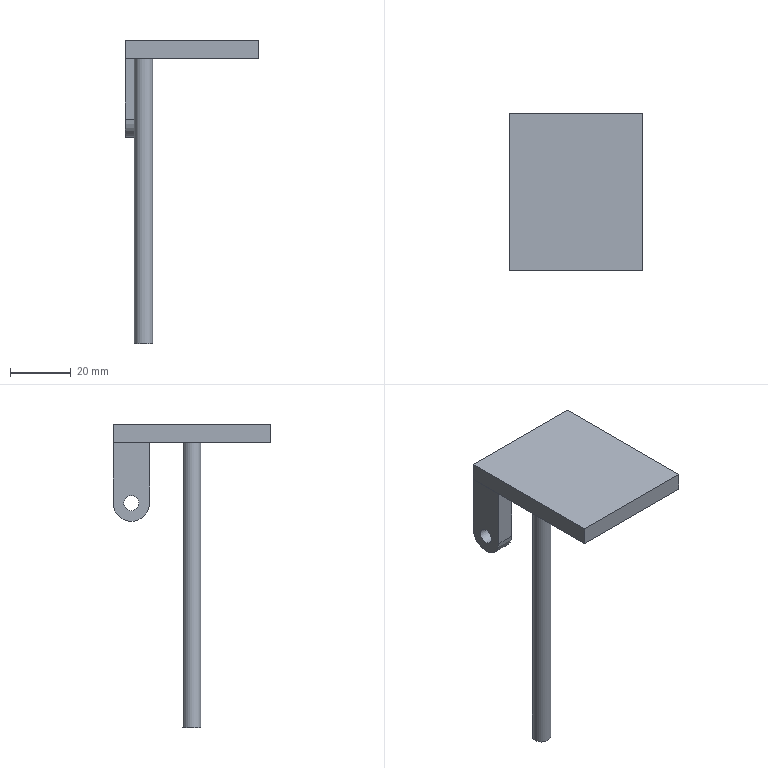Component | NX | PRINT_BLOCK | 3 solids | 16 faces | box 44 x 52.02 x 100 mm | volume 18008 mm3 | plane 13 | cylinder 3 | commonest cylinder face diameters 6 x1 12 x1 5 x1
STEP:
#1=CARTESIAN_POINT('',(0.,0.,0.));
#2=DIRECTION('',(0.,0.,1.));
#3=DIRECTION('',(1.,0.,0.));
#4=AXIS2_PLACEMENT_3D('',#1,#2,#3);
#5=CARTESIAN_POINT('',(44.,110.002,-95.515));
#6=VERTEX_POINT('',#5);
#7=CARTESIAN_POINT('',(47.,110.002,-95.515));
#8=DIRECTION('',(0.,-0.0003321,1.));
#9=DIRECTION('',(-1.,0.,0.));
#10=AXIS2_PLACEMENT_3D('',#7,#8,#9);
#11=CIRCLE('',#10,3.);
#12=CARTESIAN_POINT('',(47.,110.002,-95.515));
#13=DIRECTION('',(0.,-0.0003321,1.));
#14=DIRECTION('',(0.,-1.,-0.0003321));
#15=AXIS2_PLACEMENT_3D('',#12,#13,#14);
#16=CYLINDRICAL_SURFACE('',#15,3.);
#17=CARTESIAN_POINT('',(4.712,0.));
#18=DIRECTION('',(1.,0.));
#19=VECTOR('',#18,1.);
#20=LINE('',#17,#19);
#21=(GEOMETRIC_REPRESENTATION_CONTEXT(2)PARAMETRIC_REPRESENTATION_CONTEXT()REPRESENTATION_CONTEXT('',''));
#22=DEFINITIONAL_REPRESENTATION('',(#20),#21);
#23=PCURVE('',#16,#22);
#24=CARTESIAN_POINT('',(47.,110.002,-95.515));
#25=DIRECTION('',(0.,-0.0003321,1.));
#26=DIRECTION('',(0.,-1.,-0.0003321));
#27=AXIS2_PLACEMENT_3D('',#24,#25,#26);
#28=PLANE('',#27);
#29=CARTESIAN_POINT('',(0.,0.));
#30=DIRECTION('',(0.,-1.));
#31=AXIS2_PLACEMENT_2D('',#29,#30);
#32=CIRCLE('',#31,3.);
#33=(GEOMETRIC_REPRESENTATION_CONTEXT(2)PARAMETRIC_REPRESENTATION_CONTEXT()REPRESENTATION_CONTEXT('',''));
#34=DEFINITIONAL_REPRESENTATION('',(#32),#33);
#35=PCURVE('',#28,#34);
#36=SURFACE_CURVE('',#11,(#23,#35),.PCURVE_S1.);
#37=EDGE_CURVE('',#6,#6,#36,.T.);
#38=ORIENTED_EDGE('',*,*,#37,.T.);
#39=CARTESIAN_POINT('',(44.,109.971,-1.506));
#40=VERTEX_POINT('',#39);
#41=CARTESIAN_POINT('',(44.,110.002,-95.515));
#42=CARTESIAN_POINT('',(44.,109.971,-1.506));
#43=B_SPLINE_CURVE_WITH_KNOTS('',1,(#41,#42),.UNSPECIFIED.,.F.,.F.,(2,2),(0.,94.009),.PIECEWISE_BEZIER_KNOTS.);
#44=CARTESIAN_POINT('',(10.996,0.));
#45=DIRECTION('',(0.,1.));
#46=VECTOR('',#45,1.);
#47=LINE('',#44,#46);
#48=(GEOMETRIC_REPRESENTATION_CONTEXT(2)PARAMETRIC_REPRESENTATION_CONTEXT()REPRESENTATION_CONTEXT('',''));
#49=DEFINITIONAL_REPRESENTATION('',(#47),#48);
#50=PCURVE('',#16,#49);
#51=CARTESIAN_POINT('',(4.712,0.));
#52=DIRECTION('',(0.,1.));
#53=VECTOR('',#52,1.);
#54=LINE('',#51,#53);
#55=(GEOMETRIC_REPRESENTATION_CONTEXT(2)PARAMETRIC_REPRESENTATION_CONTEXT()REPRESENTATION_CONTEXT('',''));
#56=DEFINITIONAL_REPRESENTATION('',(#54),#55);
#57=PCURVE('',#16,#56);
#58=SEAM_CURVE('',#43,(#50,#57),.PCURVE_S1.);
#59=EDGE_CURVE('',#6,#40,#58,.T.);
#60=ORIENTED_EDGE('',*,*,#59,.T.);
#61=CARTESIAN_POINT('',(47.,109.971,-1.506));
#62=DIRECTION('',(0.,-0.0003321,1.));
#63=DIRECTION('',(-1.,0.,0.));
#64=AXIS2_PLACEMENT_3D('',#61,#62,#63);
#65=CIRCLE('',#64,3.);
#66=CARTESIAN_POINT('',(4.712,94.009));
#67=DIRECTION('',(1.,0.));
#68=VECTOR('',#67,1.);
#69=LINE('',#66,#68);
#70=(GEOMETRIC_REPRESENTATION_CONTEXT(2)PARAMETRIC_REPRESENTATION_CONTEXT()REPRESENTATION_CONTEXT('',''));
#71=DEFINITIONAL_REPRESENTATION('',(#69),#70);
#72=PCURVE('',#16,#71);
#73=CARTESIAN_POINT('',(47.,109.971,-1.506));
#74=DIRECTION('',(0.,-0.0003321,1.));
#75=DIRECTION('',(0.,-1.,-0.0003321));
#76=AXIS2_PLACEMENT_3D('',#73,#74,#75);
#77=PLANE('',#76);
#78=CARTESIAN_POINT('',(0.,0.));
#79=DIRECTION('',(0.,-1.));
#80=AXIS2_PLACEMENT_2D('',#78,#79);
#81=CIRCLE('',#80,3.);
#82=(GEOMETRIC_REPRESENTATION_CONTEXT(2)PARAMETRIC_REPRESENTATION_CONTEXT()REPRESENTATION_CONTEXT('',''));
#83=DEFINITIONAL_REPRESENTATION('',(#81),#82);
#84=PCURVE('',#77,#83);
#85=SURFACE_CURVE('',#65,(#72,#84),.PCURVE_S1.);
#86=EDGE_CURVE('',#40,#40,#85,.T.);
#87=ORIENTED_EDGE('',*,*,#86,.F.);
#88=ORIENTED_EDGE('',*,*,#59,.F.);
#89=EDGE_LOOP('',(#38,#60,#87,#88));
#90=FACE_BOUND('',#89,.T.);
#91=ADVANCED_FACE('',(#90),#16,.T.);
#92=ORIENTED_EDGE('',*,*,#37,.F.);
#93=EDGE_LOOP('',(#92));
#94=FACE_BOUND('',#93,.T.);
#95=ADVANCED_FACE('',(#94),#28,.F.);
#96=ORIENTED_EDGE('',*,*,#86,.T.);
#97=EDGE_LOOP('',(#96));
#98=FACE_BOUND('',#97,.T.);
#99=ADVANCED_FACE('',(#98),#77,.T.);
#100=CLOSED_SHELL('',(#91,#95,#99));
#101=MANIFOLD_SOLID_BREP('',#100);
#102=(LENGTH_UNIT()NAMED_UNIT(*)SI_UNIT(.MILLI.,.METRE.));
#103=UNCERTAINTY_MEASURE_WITH_UNIT(LENGTH_MEASURE(0.00001),#102,'','');
#104=(NAMED_UNIT(*)PLANE_ANGLE_UNIT()SI_UNIT($,.RADIAN.));
#105=(NAMED_UNIT(*)SI_UNIT($,.STERADIAN.)SOLID_ANGLE_UNIT());
#106=(GEOMETRIC_REPRESENTATION_CONTEXT(3)GLOBAL_UNCERTAINTY_ASSIGNED_CONTEXT((#103))GLOBAL_UNIT_ASSIGNED_CONTEXT((#102,#104,#105))REPRESENTATION_CONTEXT('',''));
#107=ADVANCED_BREP_SHAPE_REPRESENTATION('',(#4,#101),#106);
#108=CARTESIAN_POINT('',(0.,0.,0.));
#109=DIRECTION('',(0.,0.,1.));
#110=DIRECTION('',(1.,0.,0.));
#111=AXIS2_PLACEMENT_3D('',#108,#109,#110);
#112=CARTESIAN_POINT('',(0.,0.,0.));
#113=DIRECTION('',(0.,0.,1.));
#114=DIRECTION('',(1.,0.,0.));
#115=AXIS2_PLACEMENT_3D('',#112,#113,#114);
#116=CARTESIAN_POINT('',(0.,0.,0.));
#117=DIRECTION('',(0.,0.,1.));
#118=DIRECTION('',(1.,0.,0.));
#119=AXIS2_PLACEMENT_3D('',#116,#117,#118);
#120=(LENGTH_UNIT()NAMED_UNIT(*)SI_UNIT(.MILLI.,.METRE.));
#121=UNCERTAINTY_MEASURE_WITH_UNIT(LENGTH_MEASURE(0.000002),#120,'','');
#122=(NAMED_UNIT(*)PLANE_ANGLE_UNIT()SI_UNIT($,.RADIAN.));
#123=(NAMED_UNIT(*)SI_UNIT($,.STERADIAN.)SOLID_ANGLE_UNIT());
#124=(GEOMETRIC_REPRESENTATION_CONTEXT(3)GLOBAL_UNCERTAINTY_ASSIGNED_CONTEXT((#121))GLOBAL_UNIT_ASSIGNED_CONTEXT((#120,#122,#123))REPRESENTATION_CONTEXT('',''));
#125=SHAPE_REPRESENTATION('',(#4,#111,#115,#119),#124);
#126=ITEM_DEFINED_TRANSFORMATION('','',#4,#111);
#127=(REPRESENTATION_RELATIONSHIP('','',#107,#125)REPRESENTATION_RELATIONSHIP_WITH_TRANSFORMATION(#126)SHAPE_REPRESENTATION_RELATIONSHIP());
#128=CARTESIAN_POINT('',(41.,135.939,-1.497));
#129=VERTEX_POINT('',#128);
#130=CARTESIAN_POINT('',(41.,83.937,-1.515));
#131=VERTEX_POINT('',#130);
#132=CARTESIAN_POINT('',(41.,135.939,-1.497));
#133=DIRECTION('',(0.,-1.,-0.0003321));
#134=VECTOR('',#133,1.);
#135=LINE('',#132,#134);
#136=CARTESIAN_POINT('',(85.,135.939,-1.497));
#137=DIRECTION('',(0.,0.0003321,-1.));
#138=DIRECTION('',(0.,1.,0.0003321));
#139=AXIS2_PLACEMENT_3D('',#136,#137,#138);
#140=PLANE('',#139);
#141=CARTESIAN_POINT('',(0.,-44.));
#142=DIRECTION('',(-1.,0.));
#143=VECTOR('',#142,1.);
#144=LINE('',#141,#143);
#145=(GEOMETRIC_REPRESENTATION_CONTEXT(2)PARAMETRIC_REPRESENTATION_CONTEXT()REPRESENTATION_CONTEXT('',''));
#146=DEFINITIONAL_REPRESENTATION('',(#144),#145);
#147=PCURVE('',#140,#146);
#148=CARTESIAN_POINT('',(41.,199.9,58.545));
#149=DIRECTION('',(-1.,0.,0.));
#150=DIRECTION('',(0.,1.,0.0006642));
#151=AXIS2_PLACEMENT_3D('',#148,#149,#150);
#152=PLANE('',#151);
#153=CARTESIAN_POINT('',(-64.,60.));
#154=DIRECTION('',(-1.,-0.0003321));
#155=VECTOR('',#154,1.);
#156=LINE('',#153,#155);
#157=(GEOMETRIC_REPRESENTATION_CONTEXT(2)PARAMETRIC_REPRESENTATION_CONTEXT()REPRESENTATION_CONTEXT('',''));
#158=DEFINITIONAL_REPRESENTATION('',(#156),#157);
#159=PCURVE('',#152,#158);
#160=SURFACE_CURVE('',#135,(#147,#159),.PCURVE_S1.);
#161=EDGE_CURVE('',#129,#131,#160,.T.);
#162=ORIENTED_EDGE('',*,*,#161,.F.);
#163=CARTESIAN_POINT('',(85.,135.939,-1.497));
#164=VERTEX_POINT('',#163);
#165=CARTESIAN_POINT('',(85.,135.939,-1.497));
#166=DIRECTION('',(-1.,0.,0.));
#167=VECTOR('',#166,1.);
#168=LINE('',#165,#167);
#169=CARTESIAN_POINT('',(0.,0.));
#170=DIRECTION('',(0.,-1.));
#171=VECTOR('',#170,1.);
#172=LINE('',#169,#171);
#173=(GEOMETRIC_REPRESENTATION_CONTEXT(2)PARAMETRIC_REPRESENTATION_CONTEXT()REPRESENTATION_CONTEXT('',''));
#174=DEFINITIONAL_REPRESENTATION('',(#172),#173);
#175=PCURVE('',#140,#174);
#176=CARTESIAN_POINT('',(85.,135.937,4.485));
#177=DIRECTION('',(0.,1.,0.0003321));
#178=DIRECTION('',(0.,-0.0003321,1.));
#179=AXIS2_PLACEMENT_3D('',#176,#177,#178);
#180=PLANE('',#179);
#181=CARTESIAN_POINT('',(-5.983,0.));
#182=DIRECTION('',(0.,-1.));
#183=VECTOR('',#182,1.);
#184=LINE('',#181,#183);
#185=(GEOMETRIC_REPRESENTATION_CONTEXT(2)PARAMETRIC_REPRESENTATION_CONTEXT()REPRESENTATION_CONTEXT('',''));
#186=DEFINITIONAL_REPRESENTATION('',(#184),#185);
#187=PCURVE('',#180,#186);
#188=SURFACE_CURVE('',#168,(#175,#187),.PCURVE_S1.);
#189=EDGE_CURVE('',#164,#129,#188,.T.);
#190=ORIENTED_EDGE('',*,*,#189,.F.);
#191=CARTESIAN_POINT('',(85.,83.937,-1.515));
#192=VERTEX_POINT('',#191);
#193=CARTESIAN_POINT('',(85.,135.939,-1.497));
#194=DIRECTION('',(0.,-1.,-0.0003321));
#195=VECTOR('',#194,1.);
#196=LINE('',#193,#195);
#197=CARTESIAN_POINT('',(0.,0.));
#198=DIRECTION('',(-1.,0.));
#199=VECTOR('',#198,1.);
#200=LINE('',#197,#199);
#201=(GEOMETRIC_REPRESENTATION_CONTEXT(2)PARAMETRIC_REPRESENTATION_CONTEXT()REPRESENTATION_CONTEXT('',''));
#202=DEFINITIONAL_REPRESENTATION('',(#200),#201);
#203=PCURVE('',#140,#202);
#204=CARTESIAN_POINT('',(85.,199.9,58.545));
#205=DIRECTION('',(-1.,0.,0.));
#206=DIRECTION('',(0.,1.,0.0006642));
#207=AXIS2_PLACEMENT_3D('',#204,#205,#206);
#208=PLANE('',#207);
#209=CARTESIAN_POINT('',(-64.,60.));
#210=DIRECTION('',(-1.,-0.0003321));
#211=VECTOR('',#210,1.);
#212=LINE('',#209,#211);
#213=(GEOMETRIC_REPRESENTATION_CONTEXT(2)PARAMETRIC_REPRESENTATION_CONTEXT()REPRESENTATION_CONTEXT('',''));
#214=DEFINITIONAL_REPRESENTATION('',(#212),#213);
#215=PCURVE('',#208,#214);
#216=SURFACE_CURVE('',#196,(#203,#215),.PCURVE_S1.);
#217=EDGE_CURVE('',#164,#192,#216,.T.);
#218=ORIENTED_EDGE('',*,*,#217,.T.);
#219=CARTESIAN_POINT('',(85.,83.937,-1.515));
#220=DIRECTION('',(-1.,0.,0.));
#221=VECTOR('',#220,1.);
#222=LINE('',#219,#221);
#223=CARTESIAN_POINT('',(-52.002,0.));
#224=DIRECTION('',(0.,-1.));
#225=VECTOR('',#224,1.);
#226=LINE('',#223,#225);
#227=(GEOMETRIC_REPRESENTATION_CONTEXT(2)PARAMETRIC_REPRESENTATION_CONTEXT()REPRESENTATION_CONTEXT('',''));
#228=DEFINITIONAL_REPRESENTATION('',(#226),#227);
#229=PCURVE('',#140,#228);
#230=CARTESIAN_POINT('',(85.,83.937,-1.515));
#231=DIRECTION('',(0.,-1.,-0.0003321));
#232=DIRECTION('',(0.,0.0003321,-1.));
#233=AXIS2_PLACEMENT_3D('',#230,#231,#232);
#234=PLANE('',#233);
#235=CARTESIAN_POINT('',(0.,0.));
#236=DIRECTION('',(0.,-1.));
#237=VECTOR('',#236,1.);
#238=LINE('',#235,#237);
#239=(GEOMETRIC_REPRESENTATION_CONTEXT(2)PARAMETRIC_REPRESENTATION_CONTEXT()REPRESENTATION_CONTEXT('',''));
#240=DEFINITIONAL_REPRESENTATION('',(#238),#239);
#241=PCURVE('',#234,#240);
#242=SURFACE_CURVE('',#222,(#229,#241),.PCURVE_S1.);
#243=EDGE_CURVE('',#192,#131,#242,.T.);
#244=ORIENTED_EDGE('',*,*,#243,.T.);
#245=EDGE_LOOP('',(#162,#190,#218,#244));
#246=FACE_BOUND('',#245,.T.);
#247=ADVANCED_FACE('',(#246),#140,.T.);
#248=CARTESIAN_POINT('',(41.,83.935,4.468));
#249=VERTEX_POINT('',#248);
#250=CARTESIAN_POINT('',(41.,83.937,-1.515));
#251=DIRECTION('',(0.,-0.0003321,1.));
#252=VECTOR('',#251,1.);
#253=LINE('',#250,#252);
#254=CARTESIAN_POINT('',(0.,-44.));
#255=DIRECTION('',(-1.,0.));
#256=VECTOR('',#255,1.);
#257=LINE('',#254,#256);
#258=(GEOMETRIC_REPRESENTATION_CONTEXT(2)PARAMETRIC_REPRESENTATION_CONTEXT()REPRESENTATION_CONTEXT('',''));
#259=DEFINITIONAL_REPRESENTATION('',(#257),#258);
#260=PCURVE('',#234,#259);
#261=CARTESIAN_POINT('',(-116.002,59.983));
#262=DIRECTION('',(0.0003321,-1.));
#263=VECTOR('',#262,1.);
#264=LINE('',#261,#263);
#265=(GEOMETRIC_REPRESENTATION_CONTEXT(2)PARAMETRIC_REPRESENTATION_CONTEXT()REPRESENTATION_CONTEXT('',''));
#266=DEFINITIONAL_REPRESENTATION('',(#264),#265);
#267=PCURVE('',#152,#266);
#268=SURFACE_CURVE('',#253,(#260,#267),.PCURVE_S1.);
#269=EDGE_CURVE('',#131,#249,#268,.T.);
#270=ORIENTED_EDGE('',*,*,#269,.F.);
#271=ORIENTED_EDGE('',*,*,#243,.F.);
#272=CARTESIAN_POINT('',(85.,83.935,4.468));
#273=VERTEX_POINT('',#272);
#274=CARTESIAN_POINT('',(85.,83.937,-1.515));
#275=DIRECTION('',(0.,-0.0003321,1.));
#276=VECTOR('',#275,1.);
#277=LINE('',#274,#276);
#278=CARTESIAN_POINT('',(0.,0.));
#279=DIRECTION('',(-1.,0.));
#280=VECTOR('',#279,1.);
#281=LINE('',#278,#280);
#282=(GEOMETRIC_REPRESENTATION_CONTEXT(2)PARAMETRIC_REPRESENTATION_CONTEXT()REPRESENTATION_CONTEXT('',''));
#283=DEFINITIONAL_REPRESENTATION('',(#281),#282);
#284=PCURVE('',#234,#283);
#285=CARTESIAN_POINT('',(-116.002,59.983));
#286=DIRECTION('',(0.0003321,-1.));
#287=VECTOR('',#286,1.);
#288=LINE('',#285,#287);
#289=(GEOMETRIC_REPRESENTATION_CONTEXT(2)PARAMETRIC_REPRESENTATION_CONTEXT()REPRESENTATION_CONTEXT('',''));
#290=DEFINITIONAL_REPRESENTATION('',(#288),#289);
#291=PCURVE('',#208,#290);
#292=SURFACE_CURVE('',#277,(#284,#291),.PCURVE_S1.);
#293=EDGE_CURVE('',#192,#273,#292,.T.);
#294=ORIENTED_EDGE('',*,*,#293,.T.);
#295=CARTESIAN_POINT('',(85.,83.935,4.468));
#296=DIRECTION('',(-1.,0.,0.));
#297=VECTOR('',#296,1.);
#298=LINE('',#295,#297);
#299=CARTESIAN_POINT('',(-5.983,0.));
#300=DIRECTION('',(0.,-1.));
#301=VECTOR('',#300,1.);
#302=LINE('',#299,#301);
#303=(GEOMETRIC_REPRESENTATION_CONTEXT(2)PARAMETRIC_REPRESENTATION_CONTEXT()REPRESENTATION_CONTEXT('',''));
#304=DEFINITIONAL_REPRESENTATION('',(#302),#303);
#305=PCURVE('',#234,#304);
#306=CARTESIAN_POINT('',(85.,83.935,4.468));
#307=DIRECTION('',(0.,-0.0003321,1.));
#308=DIRECTION('',(0.,-1.,-0.0003321));
#309=AXIS2_PLACEMENT_3D('',#306,#307,#308);
#310=PLANE('',#309);
#311=CARTESIAN_POINT('',(0.,0.));
#312=DIRECTION('',(0.,-1.));
#313=VECTOR('',#312,1.);
#314=LINE('',#311,#313);
#315=(GEOMETRIC_REPRESENTATION_CONTEXT(2)PARAMETRIC_REPRESENTATION_CONTEXT()REPRESENTATION_CONTEXT('',''));
#316=DEFINITIONAL_REPRESENTATION('',(#314),#315);
#317=PCURVE('',#310,#316);
#318=SURFACE_CURVE('',#298,(#305,#317),.PCURVE_S1.);
#319=EDGE_CURVE('',#273,#249,#318,.T.);
#320=ORIENTED_EDGE('',*,*,#319,.T.);
#321=EDGE_LOOP('',(#270,#271,#294,#320));
#322=FACE_BOUND('',#321,.T.);
#323=ADVANCED_FACE('',(#322),#234,.T.);
#324=CARTESIAN_POINT('',(41.,135.937,4.485));
#325=VERTEX_POINT('',#324);
#326=CARTESIAN_POINT('',(41.,83.935,4.468));
#327=DIRECTION('',(0.,1.,0.0003321));
#328=VECTOR('',#327,1.);
#329=LINE('',#326,#328);
#330=CARTESIAN_POINT('',(0.,-44.));
#331=DIRECTION('',(-1.,0.));
#332=VECTOR('',#331,1.);
#333=LINE('',#330,#332);
#334=(GEOMETRIC_REPRESENTATION_CONTEXT(2)PARAMETRIC_REPRESENTATION_CONTEXT()REPRESENTATION_CONTEXT('',''));
#335=DEFINITIONAL_REPRESENTATION('',(#333),#334);
#336=PCURVE('',#310,#335);
#337=CARTESIAN_POINT('',(-116.,54.));
#338=DIRECTION('',(1.,0.0003321));
#339=VECTOR('',#338,1.);
#340=LINE('',#337,#339);
#341=(GEOMETRIC_REPRESENTATION_CONTEXT(2)PARAMETRIC_REPRESENTATION_CONTEXT()REPRESENTATION_CONTEXT('',''));
#342=DEFINITIONAL_REPRESENTATION('',(#340),#341);
#343=PCURVE('',#152,#342);
#344=SURFACE_CURVE('',#329,(#336,#343),.PCURVE_S1.);
#345=EDGE_CURVE('',#249,#325,#344,.T.);
#346=ORIENTED_EDGE('',*,*,#345,.F.);
#347=ORIENTED_EDGE('',*,*,#319,.F.);
#348=CARTESIAN_POINT('',(85.,135.937,4.485));
#349=VERTEX_POINT('',#348);
#350=CARTESIAN_POINT('',(85.,83.935,4.468));
#351=DIRECTION('',(0.,1.,0.0003321));
#352=VECTOR('',#351,1.);
#353=LINE('',#350,#352);
#354=CARTESIAN_POINT('',(0.,0.));
#355=DIRECTION('',(-1.,0.));
#356=VECTOR('',#355,1.);
#357=LINE('',#354,#356);
#358=(GEOMETRIC_REPRESENTATION_CONTEXT(2)PARAMETRIC_REPRESENTATION_CONTEXT()REPRESENTATION_CONTEXT('',''));
#359=DEFINITIONAL_REPRESENTATION('',(#357),#358);
#360=PCURVE('',#310,#359);
#361=CARTESIAN_POINT('',(-116.,54.));
#362=DIRECTION('',(1.,0.0003321));
#363=VECTOR('',#362,1.);
#364=LINE('',#361,#363);
#365=(GEOMETRIC_REPRESENTATION_CONTEXT(2)PARAMETRIC_REPRESENTATION_CONTEXT()REPRESENTATION_CONTEXT('',''));
#366=DEFINITIONAL_REPRESENTATION('',(#364),#365);
#367=PCURVE('',#208,#366);
#368=SURFACE_CURVE('',#353,(#360,#367),.PCURVE_S1.);
#369=EDGE_CURVE('',#273,#349,#368,.T.);
#370=ORIENTED_EDGE('',*,*,#369,.T.);
#371=CARTESIAN_POINT('',(85.,135.937,4.485));
#372=DIRECTION('',(-1.,0.,0.));
#373=VECTOR('',#372,1.);
#374=LINE('',#371,#373);
#375=CARTESIAN_POINT('',(-52.002,0.));
#376=DIRECTION('',(0.,-1.));
#377=VECTOR('',#376,1.);
#378=LINE('',#375,#377);
#379=(GEOMETRIC_REPRESENTATION_CONTEXT(2)PARAMETRIC_REPRESENTATION_CONTEXT()REPRESENTATION_CONTEXT('',''));
#380=DEFINITIONAL_REPRESENTATION('',(#378),#379);
#381=PCURVE('',#310,#380);
#382=CARTESIAN_POINT('',(0.,0.));
#383=DIRECTION('',(0.,-1.));
#384=VECTOR('',#383,1.);
#385=LINE('',#382,#384);
#386=(GEOMETRIC_REPRESENTATION_CONTEXT(2)PARAMETRIC_REPRESENTATION_CONTEXT()REPRESENTATION_CONTEXT('',''));
#387=DEFINITIONAL_REPRESENTATION('',(#385),#386);
#388=PCURVE('',#180,#387);
#389=SURFACE_CURVE('',#374,(#381,#388),.PCURVE_S1.);
#390=EDGE_CURVE('',#349,#325,#389,.T.);
#391=ORIENTED_EDGE('',*,*,#390,.T.);
#392=EDGE_LOOP('',(#346,#347,#370,#391));
#393=FACE_BOUND('',#392,.T.);
#394=ADVANCED_FACE('',(#393),#310,.T.);
#395=CARTESIAN_POINT('',(41.,135.937,4.485));
#396=DIRECTION('',(0.,0.0003321,-1.));
#397=VECTOR('',#396,1.);
#398=LINE('',#395,#397);
#399=CARTESIAN_POINT('',(0.,-44.));
#400=DIRECTION('',(-1.,0.));
#401=VECTOR('',#400,1.);
#402=LINE('',#399,#401);
#403=(GEOMETRIC_REPRESENTATION_CONTEXT(2)PARAMETRIC_REPRESENTATION_CONTEXT()REPRESENTATION_CONTEXT('',''));
#404=DEFINITIONAL_REPRESENTATION('',(#402),#403);
#405=PCURVE('',#180,#404);
#406=CARTESIAN_POINT('',(-63.998,54.017));
#407=DIRECTION('',(-0.0003321,1.));
#408=VECTOR('',#407,1.);
#409=LINE('',#406,#408);
#410=(GEOMETRIC_REPRESENTATION_CONTEXT(2)PARAMETRIC_REPRESENTATION_CONTEXT()REPRESENTATION_CONTEXT('',''));
#411=DEFINITIONAL_REPRESENTATION('',(#409),#410);
#412=PCURVE('',#152,#411);
#413=SURFACE_CURVE('',#398,(#405,#412),.PCURVE_S1.);
#414=EDGE_CURVE('',#325,#129,#413,.T.);
#415=ORIENTED_EDGE('',*,*,#414,.F.);
#416=ORIENTED_EDGE('',*,*,#390,.F.);
#417=CARTESIAN_POINT('',(85.,135.937,4.485));
#418=DIRECTION('',(0.,0.0003321,-1.));
#419=VECTOR('',#418,1.);
#420=LINE('',#417,#419);
#421=CARTESIAN_POINT('',(0.,0.));
#422=DIRECTION('',(-1.,0.));
#423=VECTOR('',#422,1.);
#424=LINE('',#421,#423);
#425=(GEOMETRIC_REPRESENTATION_CONTEXT(2)PARAMETRIC_REPRESENTATION_CONTEXT()REPRESENTATION_CONTEXT('',''));
#426=DEFINITIONAL_REPRESENTATION('',(#424),#425);
#427=PCURVE('',#180,#426);
#428=CARTESIAN_POINT('',(-63.998,54.017));
#429=DIRECTION('',(-0.0003321,1.));
#430=VECTOR('',#429,1.);
#431=LINE('',#428,#430);
#432=(GEOMETRIC_REPRESENTATION_CONTEXT(2)PARAMETRIC_REPRESENTATION_CONTEXT()REPRESENTATION_CONTEXT('',''));
#433=DEFINITIONAL_REPRESENTATION('',(#431),#432);
#434=PCURVE('',#208,#433);
#435=SURFACE_CURVE('',#420,(#427,#434),.PCURVE_S1.);
#436=EDGE_CURVE('',#349,#164,#435,.T.);
#437=ORIENTED_EDGE('',*,*,#436,.T.);
#438=ORIENTED_EDGE('',*,*,#189,.T.);
#439=EDGE_LOOP('',(#415,#416,#437,#438));
#440=FACE_BOUND('',#439,.T.);
#441=ADVANCED_FACE('',(#440),#180,.T.);
#442=ORIENTED_EDGE('',*,*,#217,.F.);
#443=ORIENTED_EDGE('',*,*,#436,.F.);
#444=ORIENTED_EDGE('',*,*,#369,.F.);
#445=ORIENTED_EDGE('',*,*,#293,.F.);
#446=EDGE_LOOP('',(#442,#443,#444,#445));
#447=FACE_BOUND('',#446,.T.);
#448=ADVANCED_FACE('',(#447),#208,.F.);
#449=ORIENTED_EDGE('',*,*,#161,.T.);
#450=ORIENTED_EDGE('',*,*,#269,.T.);
#451=ORIENTED_EDGE('',*,*,#345,.T.);
#452=ORIENTED_EDGE('',*,*,#414,.T.);
#453=EDGE_LOOP('',(#449,#450,#451,#452));
#454=FACE_BOUND('',#453,.T.);
#455=ADVANCED_FACE('',(#454),#152,.T.);
#456=CLOSED_SHELL('',(#247,#323,#394,#441,#448,#455));
#457=MANIFOLD_SOLID_BREP('',#456);
#458=(LENGTH_UNIT()NAMED_UNIT(*)SI_UNIT(.MILLI.,.METRE.));
#459=UNCERTAINTY_MEASURE_WITH_UNIT(LENGTH_MEASURE(0.0000001),#458,'','');
#460=(NAMED_UNIT(*)PLANE_ANGLE_UNIT()SI_UNIT($,.RADIAN.));
#461=(NAMED_UNIT(*)SI_UNIT($,.STERADIAN.)SOLID_ANGLE_UNIT());
#462=(GEOMETRIC_REPRESENTATION_CONTEXT(3)GLOBAL_UNCERTAINTY_ASSIGNED_CONTEXT((#459))GLOBAL_UNIT_ASSIGNED_CONTEXT((#458,#460,#461))REPRESENTATION_CONTEXT('',''));
#463=ADVANCED_BREP_SHAPE_REPRESENTATION('',(#4,#457),#462);
#464=ITEM_DEFINED_TRANSFORMATION('','',#4,#115);
#465=(REPRESENTATION_RELATIONSHIP('','',#463,#125)REPRESENTATION_RELATIONSHIP_WITH_TRANSFORMATION(#464)SHAPE_REPRESENTATION_RELATIONSHIP());
#466=CARTESIAN_POINT('',(47.,135.946,-21.217));
#467=VERTEX_POINT('',#466);
#468=CARTESIAN_POINT('',(47.,123.953,-21.501));
#469=VERTEX_POINT('',#468);
#470=CARTESIAN_POINT('',(47.,129.953,-21.501));
#471=DIRECTION('',(-1.,0.,0.));
#472=DIRECTION('',(0.,0.0003321,-1.));
#473=AXIS2_PLACEMENT_3D('',#470,#471,#472);
#474=CIRCLE('',#473,6.);
#475=CARTESIAN_POINT('',(41.,129.953,-21.501));
#476=DIRECTION('',(1.,0.,0.));
#477=DIRECTION('',(0.,-1.,-0.0006642));
#478=AXIS2_PLACEMENT_3D('',#475,#476,#477);
#479=CYLINDRICAL_SURFACE('',#478,6.);
#480=CARTESIAN_POINT('',(7.854,6.));
#481=DIRECTION('',(-1.,0.));
#482=VECTOR('',#481,1.);
#483=LINE('',#480,#482);
#484=(GEOMETRIC_REPRESENTATION_CONTEXT(2)PARAMETRIC_REPRESENTATION_CONTEXT()REPRESENTATION_CONTEXT('',''));
#485=DEFINITIONAL_REPRESENTATION('',(#483),#484);
#486=PCURVE('',#479,#485);
#487=CARTESIAN_POINT('',(47.,129.953,-21.501));
#488=DIRECTION('',(-1.,0.,0.));
#489=DIRECTION('',(0.,1.,0.0006642));
#490=AXIS2_PLACEMENT_3D('',#487,#488,#489);
#491=PLANE('',#490);
#492=CARTESIAN_POINT('',(0.,0.));
#493=DIRECTION('',(-0.0003321,1.));
#494=AXIS2_PLACEMENT_2D('',#492,#493);
#495=CIRCLE('',#494,6.);
#496=(GEOMETRIC_REPRESENTATION_CONTEXT(2)PARAMETRIC_REPRESENTATION_CONTEXT()REPRESENTATION_CONTEXT('',''));
#497=DEFINITIONAL_REPRESENTATION('',(#495),#496);
#498=PCURVE('',#491,#497);
#499=SURFACE_CURVE('',#474,(#486,#498),.PCURVE_S1.);
#500=EDGE_CURVE('',#467,#469,#499,.T.);
#501=ORIENTED_EDGE('',*,*,#500,.T.);
#502=CARTESIAN_POINT('',(41.,123.953,-21.501));
#503=VERTEX_POINT('',#502);
#504=CARTESIAN_POINT('',(41.,123.953,-21.501));
#505=DIRECTION('',(1.,0.,0.));
#506=VECTOR('',#505,1.);
#507=LINE('',#504,#506);
#508=CARTESIAN_POINT('',(-0.0006903,0.));
#509=DIRECTION('',(0.,1.));
#510=VECTOR('',#509,1.);
#511=LINE('',#508,#510);
#512=(GEOMETRIC_REPRESENTATION_CONTEXT(2)PARAMETRIC_REPRESENTATION_CONTEXT()REPRESENTATION_CONTEXT('',''));
#513=DEFINITIONAL_REPRESENTATION('',(#511),#512);
#514=PCURVE('',#479,#513);
#515=CARTESIAN_POINT('',(41.,123.953,-21.501));
#516=DIRECTION('',(0.,1.,0.0003321));
#517=DIRECTION('',(0.,-0.0003321,1.));
#518=AXIS2_PLACEMENT_3D('',#515,#516,#517);
#519=PLANE('',#518);
#520=CARTESIAN_POINT('',(-0.,0.));
#521=DIRECTION('',(0.,1.));
#522=VECTOR('',#521,1.);
#523=LINE('',#520,#522);
#524=(GEOMETRIC_REPRESENTATION_CONTEXT(2)PARAMETRIC_REPRESENTATION_CONTEXT()REPRESENTATION_CONTEXT('',''));
#525=DEFINITIONAL_REPRESENTATION('',(#523),#524);
#526=PCURVE('',#519,#525);
#527=SURFACE_CURVE('',#507,(#514,#526),.PCURVE_S1.);
#528=EDGE_CURVE('',#503,#469,#527,.T.);
#529=ORIENTED_EDGE('',*,*,#528,.F.);
#530=CARTESIAN_POINT('',(41.,135.946,-21.217));
#531=VERTEX_POINT('',#530);
#532=CARTESIAN_POINT('',(41.,129.953,-21.501));
#533=DIRECTION('',(-1.,0.,0.));
#534=DIRECTION('',(0.,0.0003321,-1.));
#535=AXIS2_PLACEMENT_3D('',#532,#533,#534);
#536=CIRCLE('',#535,6.);
#537=CARTESIAN_POINT('',(7.854,0.));
#538=DIRECTION('',(-1.,0.));
#539=VECTOR('',#538,1.);
#540=LINE('',#537,#539);
#541=(GEOMETRIC_REPRESENTATION_CONTEXT(2)PARAMETRIC_REPRESENTATION_CONTEXT()REPRESENTATION_CONTEXT('',''));
#542=DEFINITIONAL_REPRESENTATION('',(#540),#541);
#543=PCURVE('',#479,#542);
#544=CARTESIAN_POINT('',(41.,129.953,-21.501));
#545=DIRECTION('',(-1.,0.,0.));
#546=DIRECTION('',(0.,1.,0.0006642));
#547=AXIS2_PLACEMENT_3D('',#544,#545,#546);
#548=PLANE('',#547);
#549=CARTESIAN_POINT('',(0.,0.));
#550=DIRECTION('',(-0.0003321,1.));
#551=AXIS2_PLACEMENT_2D('',#549,#550);
#552=CIRCLE('',#551,6.);
#553=(GEOMETRIC_REPRESENTATION_CONTEXT(2)PARAMETRIC_REPRESENTATION_CONTEXT()REPRESENTATION_CONTEXT('',''));
#554=DEFINITIONAL_REPRESENTATION('',(#552),#553);
#555=PCURVE('',#548,#554);
#556=SURFACE_CURVE('',#536,(#543,#555),.PCURVE_S1.);
#557=EDGE_CURVE('',#531,#503,#556,.T.);
#558=ORIENTED_EDGE('',*,*,#557,.F.);
#559=CARTESIAN_POINT('',(41.,135.946,-21.217));
#560=DIRECTION('',(1.,0.,0.));
#561=VECTOR('',#560,1.);
#562=LINE('',#559,#561);
#563=CARTESIAN_POINT('',(3.188,0.));
#564=DIRECTION('',(0.,1.));
#565=VECTOR('',#564,1.);
#566=LINE('',#563,#565);
#567=(GEOMETRIC_REPRESENTATION_CONTEXT(2)PARAMETRIC_REPRESENTATION_CONTEXT()REPRESENTATION_CONTEXT('',''));
#568=DEFINITIONAL_REPRESENTATION('',(#566),#567);
#569=PCURVE('',#479,#568);
#570=CARTESIAN_POINT('',(41.,135.939,-1.497));
#571=DIRECTION('',(0.,-1.,-0.0003321));
#572=DIRECTION('',(0.,0.0003321,-1.));
#573=AXIS2_PLACEMENT_3D('',#570,#571,#572);
#574=PLANE('',#573);
#575=CARTESIAN_POINT('',(19.72,0.));
#576=DIRECTION('',(0.,1.));
#577=VECTOR('',#576,1.);
#578=LINE('',#575,#577);
#579=(GEOMETRIC_REPRESENTATION_CONTEXT(2)PARAMETRIC_REPRESENTATION_CONTEXT()REPRESENTATION_CONTEXT('',''));
#580=DEFINITIONAL_REPRESENTATION('',(#578),#579);
#581=PCURVE('',#574,#580);
#582=SURFACE_CURVE('',#562,(#569,#581),.PCURVE_S1.);
#583=EDGE_CURVE('',#531,#467,#582,.T.);
#584=ORIENTED_EDGE('',*,*,#583,.T.);
#585=EDGE_LOOP('',(#501,#529,#558,#584));
#586=FACE_BOUND('',#585,.T.);
#587=ADVANCED_FACE('',(#586),#479,.T.);
#588=CARTESIAN_POINT('',(47.,123.946,-1.501));
#589=VERTEX_POINT('',#588);
#590=CARTESIAN_POINT('',(47.,123.953,-21.501));
#591=DIRECTION('',(0.,-0.0003321,1.));
#592=VECTOR('',#591,1.);
#593=LINE('',#590,#592);
#594=CARTESIAN_POINT('',(0.,6.));
#595=DIRECTION('',(1.,0.));
#596=VECTOR('',#595,1.);
#597=LINE('',#594,#596);
#598=(GEOMETRIC_REPRESENTATION_CONTEXT(2)PARAMETRIC_REPRESENTATION_CONTEXT()REPRESENTATION_CONTEXT('',''));
#599=DEFINITIONAL_REPRESENTATION('',(#597),#598);
#600=PCURVE('',#519,#599);
#601=CARTESIAN_POINT('',(-6.,-0.004142));
#602=DIRECTION('',(0.0003321,-1.));
#603=VECTOR('',#602,1.);
#604=LINE('',#601,#603);
#605=(GEOMETRIC_REPRESENTATION_CONTEXT(2)PARAMETRIC_REPRESENTATION_CONTEXT()REPRESENTATION_CONTEXT('',''));
#606=DEFINITIONAL_REPRESENTATION('',(#604),#605);
#607=PCURVE('',#491,#606);
#608=SURFACE_CURVE('',#593,(#600,#607),.PCURVE_S1.);
#609=EDGE_CURVE('',#469,#589,#608,.T.);
#610=ORIENTED_EDGE('',*,*,#609,.T.);
#611=CARTESIAN_POINT('',(41.,123.946,-1.501));
#612=VERTEX_POINT('',#611);
#613=CARTESIAN_POINT('',(41.,123.946,-1.501));
#614=DIRECTION('',(1.,0.,0.));
#615=VECTOR('',#614,1.);
#616=LINE('',#613,#615);
#617=CARTESIAN_POINT('',(20.,0.));
#618=DIRECTION('',(0.,1.));
#619=VECTOR('',#618,1.);
#620=LINE('',#617,#619);
#621=(GEOMETRIC_REPRESENTATION_CONTEXT(2)PARAMETRIC_REPRESENTATION_CONTEXT()REPRESENTATION_CONTEXT('',''));
#622=DEFINITIONAL_REPRESENTATION('',(#620),#621);
#623=PCURVE('',#519,#622);
#624=CARTESIAN_POINT('',(41.,123.946,-1.501));
#625=DIRECTION('',(0.,0.0003321,-1.));
#626=DIRECTION('',(0.,1.,0.0003321));
#627=AXIS2_PLACEMENT_3D('',#624,#625,#626);
#628=PLANE('',#627);
#629=CARTESIAN_POINT('',(0.,0.));
#630=DIRECTION('',(0.,1.));
#631=VECTOR('',#630,1.);
#632=LINE('',#629,#631);
#633=(GEOMETRIC_REPRESENTATION_CONTEXT(2)PARAMETRIC_REPRESENTATION_CONTEXT()REPRESENTATION_CONTEXT('',''));
#634=DEFINITIONAL_REPRESENTATION('',(#632),#633);
#635=PCURVE('',#628,#634);
#636=SURFACE_CURVE('',#616,(#623,#635),.PCURVE_S1.);
#637=EDGE_CURVE('',#612,#589,#636,.T.);
#638=ORIENTED_EDGE('',*,*,#637,.F.);
#639=CARTESIAN_POINT('',(41.,123.953,-21.501));
#640=DIRECTION('',(0.,-0.0003321,1.));
#641=VECTOR('',#640,1.);
#642=LINE('',#639,#641);
#643=CARTESIAN_POINT('',(0.,0.));
#644=DIRECTION('',(1.,0.));
#645=VECTOR('',#644,1.);
#646=LINE('',#643,#645);
#647=(GEOMETRIC_REPRESENTATION_CONTEXT(2)PARAMETRIC_REPRESENTATION_CONTEXT()REPRESENTATION_CONTEXT('',''));
#648=DEFINITIONAL_REPRESENTATION('',(#646),#647);
#649=PCURVE('',#519,#648);
#650=CARTESIAN_POINT('',(-6.,-0.004142));
#651=DIRECTION('',(0.0003321,-1.));
#652=VECTOR('',#651,1.);
#653=LINE('',#650,#652);
#654=(GEOMETRIC_REPRESENTATION_CONTEXT(2)PARAMETRIC_REPRESENTATION_CONTEXT()REPRESENTATION_CONTEXT('',''));
#655=DEFINITIONAL_REPRESENTATION('',(#653),#654);
#656=PCURVE('',#548,#655);
#657=SURFACE_CURVE('',#642,(#649,#656),.PCURVE_S1.);
#658=EDGE_CURVE('',#503,#612,#657,.T.);
#659=ORIENTED_EDGE('',*,*,#658,.F.);
#660=ORIENTED_EDGE('',*,*,#528,.T.);
#661=EDGE_LOOP('',(#610,#638,#659,#660));
#662=FACE_BOUND('',#661,.T.);
#663=ADVANCED_FACE('',(#662),#519,.F.);
#664=CARTESIAN_POINT('',(47.,135.939,-1.497));
#665=VERTEX_POINT('',#664);
#666=CARTESIAN_POINT('',(47.,123.946,-1.501));
#667=DIRECTION('',(0.,1.,0.0003321));
#668=VECTOR('',#667,1.);
#669=LINE('',#666,#668);
#670=CARTESIAN_POINT('',(0.,6.));
#671=DIRECTION('',(1.,0.));
#672=VECTOR('',#671,1.);
#673=LINE('',#670,#672);
#674=(GEOMETRIC_REPRESENTATION_CONTEXT(2)PARAMETRIC_REPRESENTATION_CONTEXT()REPRESENTATION_CONTEXT('',''));
#675=DEFINITIONAL_REPRESENTATION('',(#673),#674);
#676=PCURVE('',#628,#675);
#677=CARTESIAN_POINT('',(-5.993,-20.004));
#678=DIRECTION('',(1.,0.0003321));
#679=VECTOR('',#678,1.);
#680=LINE('',#677,#679);
#681=(GEOMETRIC_REPRESENTATION_CONTEXT(2)PARAMETRIC_REPRESENTATION_CONTEXT()REPRESENTATION_CONTEXT('',''));
#682=DEFINITIONAL_REPRESENTATION('',(#680),#681);
#683=PCURVE('',#491,#682);
#684=SURFACE_CURVE('',#669,(#676,#683),.PCURVE_S1.);
#685=EDGE_CURVE('',#589,#665,#684,.T.);
#686=ORIENTED_EDGE('',*,*,#685,.T.);
#687=CARTESIAN_POINT('',(41.,135.939,-1.497));
#688=VERTEX_POINT('',#687);
#689=CARTESIAN_POINT('',(41.,135.939,-1.497));
#690=DIRECTION('',(1.,0.,0.));
#691=VECTOR('',#690,1.);
#692=LINE('',#689,#691);
#693=CARTESIAN_POINT('',(11.993,0.));
#694=DIRECTION('',(0.,1.));
#695=VECTOR('',#694,1.);
#696=LINE('',#693,#695);
#697=(GEOMETRIC_REPRESENTATION_CONTEXT(2)PARAMETRIC_REPRESENTATION_CONTEXT()REPRESENTATION_CONTEXT('',''));
#698=DEFINITIONAL_REPRESENTATION('',(#696),#697);
#699=PCURVE('',#628,#698);
#700=CARTESIAN_POINT('',(0.,0.));
#701=DIRECTION('',(0.,1.));
#702=VECTOR('',#701,1.);
#703=LINE('',#700,#702);
#704=(GEOMETRIC_REPRESENTATION_CONTEXT(2)PARAMETRIC_REPRESENTATION_CONTEXT()REPRESENTATION_CONTEXT('',''));
#705=DEFINITIONAL_REPRESENTATION('',(#703),#704);
#706=PCURVE('',#574,#705);
#707=SURFACE_CURVE('',#692,(#699,#706),.PCURVE_S1.);
#708=EDGE_CURVE('',#688,#665,#707,.T.);
#709=ORIENTED_EDGE('',*,*,#708,.F.);
#710=CARTESIAN_POINT('',(41.,123.946,-1.501));
#711=DIRECTION('',(0.,1.,0.0003321));
#712=VECTOR('',#711,1.);
#713=LINE('',#710,#712);
#714=CARTESIAN_POINT('',(0.,0.));
#715=DIRECTION('',(1.,0.));
#716=VECTOR('',#715,1.);
#717=LINE('',#714,#716);
#718=(GEOMETRIC_REPRESENTATION_CONTEXT(2)PARAMETRIC_REPRESENTATION_CONTEXT()REPRESENTATION_CONTEXT('',''));
#719=DEFINITIONAL_REPRESENTATION('',(#717),#718);
#720=PCURVE('',#628,#719);
#721=CARTESIAN_POINT('',(-5.993,-20.004));
#722=DIRECTION('',(1.,0.0003321));
#723=VECTOR('',#722,1.);
#724=LINE('',#721,#723);
#725=(GEOMETRIC_REPRESENTATION_CONTEXT(2)PARAMETRIC_REPRESENTATION_CONTEXT()REPRESENTATION_CONTEXT('',''));
#726=DEFINITIONAL_REPRESENTATION('',(#724),#725);
#727=PCURVE('',#548,#726);
#728=SURFACE_CURVE('',#713,(#720,#727),.PCURVE_S1.);
#729=EDGE_CURVE('',#612,#688,#728,.T.);
#730=ORIENTED_EDGE('',*,*,#729,.F.);
#731=ORIENTED_EDGE('',*,*,#637,.T.);
#732=EDGE_LOOP('',(#686,#709,#730,#731));
#733=FACE_BOUND('',#732,.T.);
#734=ADVANCED_FACE('',(#733),#628,.F.);
#735=CARTESIAN_POINT('',(47.,135.939,-1.497));
#736=DIRECTION('',(0.,0.0003321,-1.));
#737=VECTOR('',#736,1.);
#738=LINE('',#735,#737);
#739=CARTESIAN_POINT('',(0.,6.));
#740=DIRECTION('',(1.,0.));
#741=VECTOR('',#740,1.);
#742=LINE('',#739,#741);
#743=(GEOMETRIC_REPRESENTATION_CONTEXT(2)PARAMETRIC_REPRESENTATION_CONTEXT()REPRESENTATION_CONTEXT('',''));
#744=DEFINITIONAL_REPRESENTATION('',(#742),#743);
#745=PCURVE('',#574,#744);
#746=CARTESIAN_POINT('',(6.,-20.));
#747=DIRECTION('',(-0.0003321,1.));
#748=VECTOR('',#747,1.);
#749=LINE('',#746,#748);
#750=(GEOMETRIC_REPRESENTATION_CONTEXT(2)PARAMETRIC_REPRESENTATION_CONTEXT()REPRESENTATION_CONTEXT('',''));
#751=DEFINITIONAL_REPRESENTATION('',(#749),#750);
#752=PCURVE('',#491,#751);
#753=SURFACE_CURVE('',#738,(#745,#752),.PCURVE_S1.);
#754=EDGE_CURVE('',#665,#467,#753,.T.);
#755=ORIENTED_EDGE('',*,*,#754,.T.);
#756=ORIENTED_EDGE('',*,*,#583,.F.);
#757=CARTESIAN_POINT('',(41.,135.939,-1.497));
#758=DIRECTION('',(0.,0.0003321,-1.));
#759=VECTOR('',#758,1.);
#760=LINE('',#757,#759);
#761=CARTESIAN_POINT('',(0.,0.));
#762=DIRECTION('',(1.,0.));
#763=VECTOR('',#762,1.);
#764=LINE('',#761,#763);
#765=(GEOMETRIC_REPRESENTATION_CONTEXT(2)PARAMETRIC_REPRESENTATION_CONTEXT()REPRESENTATION_CONTEXT('',''));
#766=DEFINITIONAL_REPRESENTATION('',(#764),#765);
#767=PCURVE('',#574,#766);
#768=CARTESIAN_POINT('',(6.,-20.));
#769=DIRECTION('',(-0.0003321,1.));
#770=VECTOR('',#769,1.);
#771=LINE('',#768,#770);
#772=(GEOMETRIC_REPRESENTATION_CONTEXT(2)PARAMETRIC_REPRESENTATION_CONTEXT()REPRESENTATION_CONTEXT('',''));
#773=DEFINITIONAL_REPRESENTATION('',(#771),#772);
#774=PCURVE('',#548,#773);
#775=SURFACE_CURVE('',#760,(#767,#774),.PCURVE_S1.);
#776=EDGE_CURVE('',#688,#531,#775,.T.);
#777=ORIENTED_EDGE('',*,*,#776,.F.);
#778=ORIENTED_EDGE('',*,*,#708,.T.);
#779=EDGE_LOOP('',(#755,#756,#777,#778));
#780=FACE_BOUND('',#779,.T.);
#781=ADVANCED_FACE('',(#780),#574,.F.);
#782=CARTESIAN_POINT('',(41.,129.954,-24.001));
#783=VERTEX_POINT('',#782);
#784=CARTESIAN_POINT('',(41.,129.953,-21.501));
#785=DIRECTION('',(1.,0.,0.));
#786=DIRECTION('',(0.,0.0003321,-1.));
#787=AXIS2_PLACEMENT_3D('',#784,#785,#786);
#788=CIRCLE('',#787,2.5);
#789=CARTESIAN_POINT('',(41.,129.953,-21.501));
#790=DIRECTION('',(1.,0.,0.));
#791=DIRECTION('',(0.,-1.,-0.0006642));
#792=AXIS2_PLACEMENT_3D('',#789,#790,#791);
#793=CYLINDRICAL_SURFACE('',#792,2.5);
#794=CARTESIAN_POINT('',(1.57,0.));
#795=DIRECTION('',(1.,0.));
#796=VECTOR('',#795,1.);
#797=LINE('',#794,#796);
#798=(GEOMETRIC_REPRESENTATION_CONTEXT(2)PARAMETRIC_REPRESENTATION_CONTEXT()REPRESENTATION_CONTEXT('',''));
#799=DEFINITIONAL_REPRESENTATION('',(#797),#798);
#800=PCURVE('',#793,#799);
#801=CARTESIAN_POINT('',(-0.0008303,2.5));
#802=CARTESIAN_POINT('',(4.329,2.501));
#803=CARTESIAN_POINT('',(2.165,-1.249));
#804=CARTESIAN_POINT('',(0.001661,-5.));
#805=CARTESIAN_POINT('',(-2.165,-1.251));
#806=CARTESIAN_POINT('',(-4.331,2.499));
#807=CARTESIAN_POINT('',(-0.0008303,2.5));
#808=(BOUNDED_CURVE()B_SPLINE_CURVE(2,(#801,#802,#803,#804,#805,#806,#807),.UNSPECIFIED.,.T.,.F.)B_SPLINE_CURVE_WITH_KNOTS((1,2,2,2,2,1),(-2.094,0.,2.094,4.189,6.283,8.378),.UNSPECIFIED.)CURVE()GEOMETRIC_REPRESENTATION_ITEM()RATIONAL_B_SPLINE_CURVE((1.,0.5,1.,0.5,1.,0.5,1.))REPRESENTATION_ITEM(''));
#809=(GEOMETRIC_REPRESENTATION_CONTEXT(2)PARAMETRIC_REPRESENTATION_CONTEXT()REPRESENTATION_CONTEXT('',''));
#810=DEFINITIONAL_REPRESENTATION('',(#808),#809);
#811=PCURVE('',#548,#810);
#812=SURFACE_CURVE('',#788,(#800,#811),.PCURVE_S1.);
#813=EDGE_CURVE('',#783,#783,#812,.T.);
#814=ORIENTED_EDGE('',*,*,#813,.T.);
#815=CARTESIAN_POINT('',(47.,129.954,-24.001));
#816=VERTEX_POINT('',#815);
#817=CARTESIAN_POINT('',(41.,129.954,-24.001));
#818=CARTESIAN_POINT('',(47.,129.954,-24.001));
#819=B_SPLINE_CURVE_WITH_KNOTS('',1,(#817,#818),.UNSPECIFIED.,.F.,.F.,(2,2),(0.,6.),.PIECEWISE_BEZIER_KNOTS.);
#820=CARTESIAN_POINT('',(7.854,0.));
#821=DIRECTION('',(0.,1.));
#822=VECTOR('',#821,1.);
#823=LINE('',#820,#822);
#824=(GEOMETRIC_REPRESENTATION_CONTEXT(2)PARAMETRIC_REPRESENTATION_CONTEXT()REPRESENTATION_CONTEXT('',''));
#825=DEFINITIONAL_REPRESENTATION('',(#823),#824);
#826=PCURVE('',#793,#825);
#827=CARTESIAN_POINT('',(1.57,0.));
#828=DIRECTION('',(0.,1.));
#829=VECTOR('',#828,1.);
#830=LINE('',#827,#829);
#831=(GEOMETRIC_REPRESENTATION_CONTEXT(2)PARAMETRIC_REPRESENTATION_CONTEXT()REPRESENTATION_CONTEXT('',''));
#832=DEFINITIONAL_REPRESENTATION('',(#830),#831);
#833=PCURVE('',#793,#832);
#834=SEAM_CURVE('',#819,(#826,#833),.PCURVE_S1.);
#835=EDGE_CURVE('',#783,#816,#834,.T.);
#836=ORIENTED_EDGE('',*,*,#835,.T.);
#837=CARTESIAN_POINT('',(47.,129.953,-21.501));
#838=DIRECTION('',(1.,0.,0.));
#839=DIRECTION('',(0.,0.0003321,-1.));
#840=AXIS2_PLACEMENT_3D('',#837,#838,#839);
#841=CIRCLE('',#840,2.5);
#842=CARTESIAN_POINT('',(1.57,6.));
#843=DIRECTION('',(1.,0.));
#844=VECTOR('',#843,1.);
#845=LINE('',#842,#844);
#846=(GEOMETRIC_REPRESENTATION_CONTEXT(2)PARAMETRIC_REPRESENTATION_CONTEXT()REPRESENTATION_CONTEXT('',''));
#847=DEFINITIONAL_REPRESENTATION('',(#845),#846);
#848=PCURVE('',#793,#847);
#849=CARTESIAN_POINT('',(-0.0008303,2.5));
#850=CARTESIAN_POINT('',(4.329,2.501));
#851=CARTESIAN_POINT('',(2.165,-1.249));
#852=CARTESIAN_POINT('',(0.001661,-5.));
#853=CARTESIAN_POINT('',(-2.165,-1.251));
#854=CARTESIAN_POINT('',(-4.331,2.499));
#855=CARTESIAN_POINT('',(-0.0008303,2.5));
#856=(BOUNDED_CURVE()B_SPLINE_CURVE(2,(#849,#850,#851,#852,#853,#854,#855),.UNSPECIFIED.,.T.,.F.)B_SPLINE_CURVE_WITH_KNOTS((1,2,2,2,2,1),(-2.094,0.,2.094,4.189,6.283,8.378),.UNSPECIFIED.)CURVE()GEOMETRIC_REPRESENTATION_ITEM()RATIONAL_B_SPLINE_CURVE((1.,0.5,1.,0.5,1.,0.5,1.))REPRESENTATION_ITEM(''));
#857=(GEOMETRIC_REPRESENTATION_CONTEXT(2)PARAMETRIC_REPRESENTATION_CONTEXT()REPRESENTATION_CONTEXT('',''));
#858=DEFINITIONAL_REPRESENTATION('',(#856),#857);
#859=PCURVE('',#491,#858);
#860=SURFACE_CURVE('',#841,(#848,#859),.PCURVE_S1.);
#861=EDGE_CURVE('',#816,#816,#860,.T.);
#862=ORIENTED_EDGE('',*,*,#861,.F.);
#863=ORIENTED_EDGE('',*,*,#835,.F.);
#864=EDGE_LOOP('',(#814,#836,#862,#863));
#865=FACE_BOUND('',#864,.F.);
#866=ADVANCED_FACE('',(#865),#793,.F.);
#867=ORIENTED_EDGE('',*,*,#557,.T.);
#868=ORIENTED_EDGE('',*,*,#658,.T.);
#869=ORIENTED_EDGE('',*,*,#729,.T.);
#870=ORIENTED_EDGE('',*,*,#776,.T.);
#871=EDGE_LOOP('',(#867,#868,#869,#870));
#872=FACE_BOUND('',#871,.T.);
#873=ORIENTED_EDGE('',*,*,#813,.T.);
#874=EDGE_LOOP('',(#873));
#875=FACE_BOUND('',#874,.T.);
#876=ADVANCED_FACE('',(#872,#875),#548,.T.);
#877=ORIENTED_EDGE('',*,*,#500,.F.);
#878=ORIENTED_EDGE('',*,*,#754,.F.);
#879=ORIENTED_EDGE('',*,*,#685,.F.);
#880=ORIENTED_EDGE('',*,*,#609,.F.);
#881=EDGE_LOOP('',(#877,#878,#879,#880));
#882=FACE_BOUND('',#881,.T.);
#883=ORIENTED_EDGE('',*,*,#861,.F.);
#884=EDGE_LOOP('',(#883));
#885=FACE_BOUND('',#884,.T.);
#886=ADVANCED_FACE('',(#882,#885),#491,.F.);
#887=CLOSED_SHELL('',(#587,#663,#734,#781,#866,#876,#886));
#888=MANIFOLD_SOLID_BREP('',#887);
#889=(LENGTH_UNIT()NAMED_UNIT(*)SI_UNIT(.MILLI.,.METRE.));
#890=UNCERTAINTY_MEASURE_WITH_UNIT(LENGTH_MEASURE(0.000002),#889,'','');
#891=(NAMED_UNIT(*)PLANE_ANGLE_UNIT()SI_UNIT($,.RADIAN.));
#892=(NAMED_UNIT(*)SI_UNIT($,.STERADIAN.)SOLID_ANGLE_UNIT());
#893=(GEOMETRIC_REPRESENTATION_CONTEXT(3)GLOBAL_UNCERTAINTY_ASSIGNED_CONTEXT((#890))GLOBAL_UNIT_ASSIGNED_CONTEXT((#889,#891,#892))REPRESENTATION_CONTEXT('',''));
#894=ADVANCED_BREP_SHAPE_REPRESENTATION('',(#4,#888),#893);
#895=ITEM_DEFINED_TRANSFORMATION('','',#4,#119);
#896=(REPRESENTATION_RELATIONSHIP('','',#894,#125)REPRESENTATION_RELATIONSHIP_WITH_TRANSFORMATION(#895)SHAPE_REPRESENTATION_RELATIONSHIP());